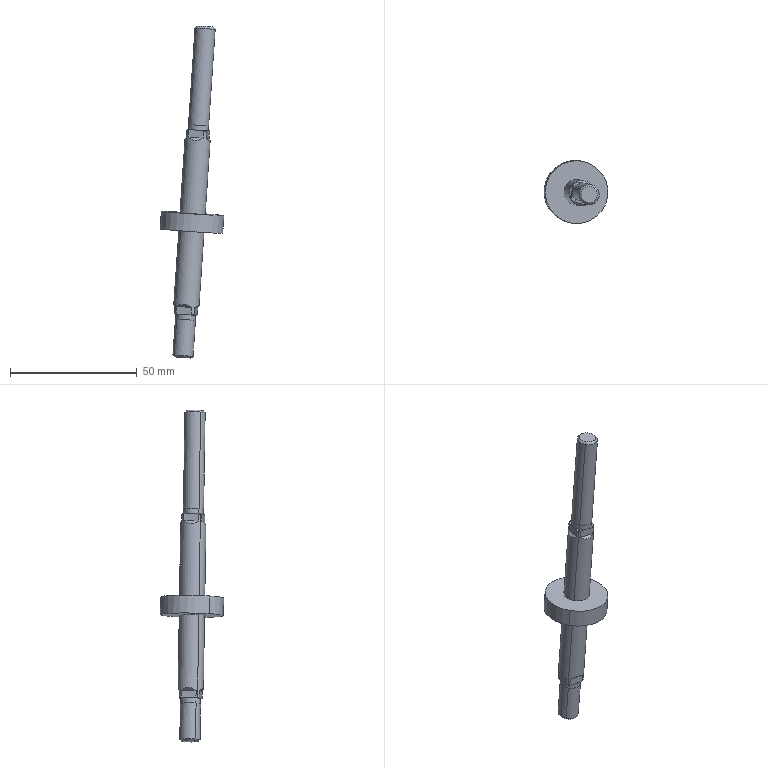Component | SolidWorks | SDAJ25x20-20B(00)+()-1_SDAJ-25x20-B2020_r-1 | 1 solid | 52 faces | volume 11372 mm3 | plane 24 | cylinder 14 | cone 14 | commonest cylinder face diameters 10 x4 7.8 x4 8 x4 24.9 x2